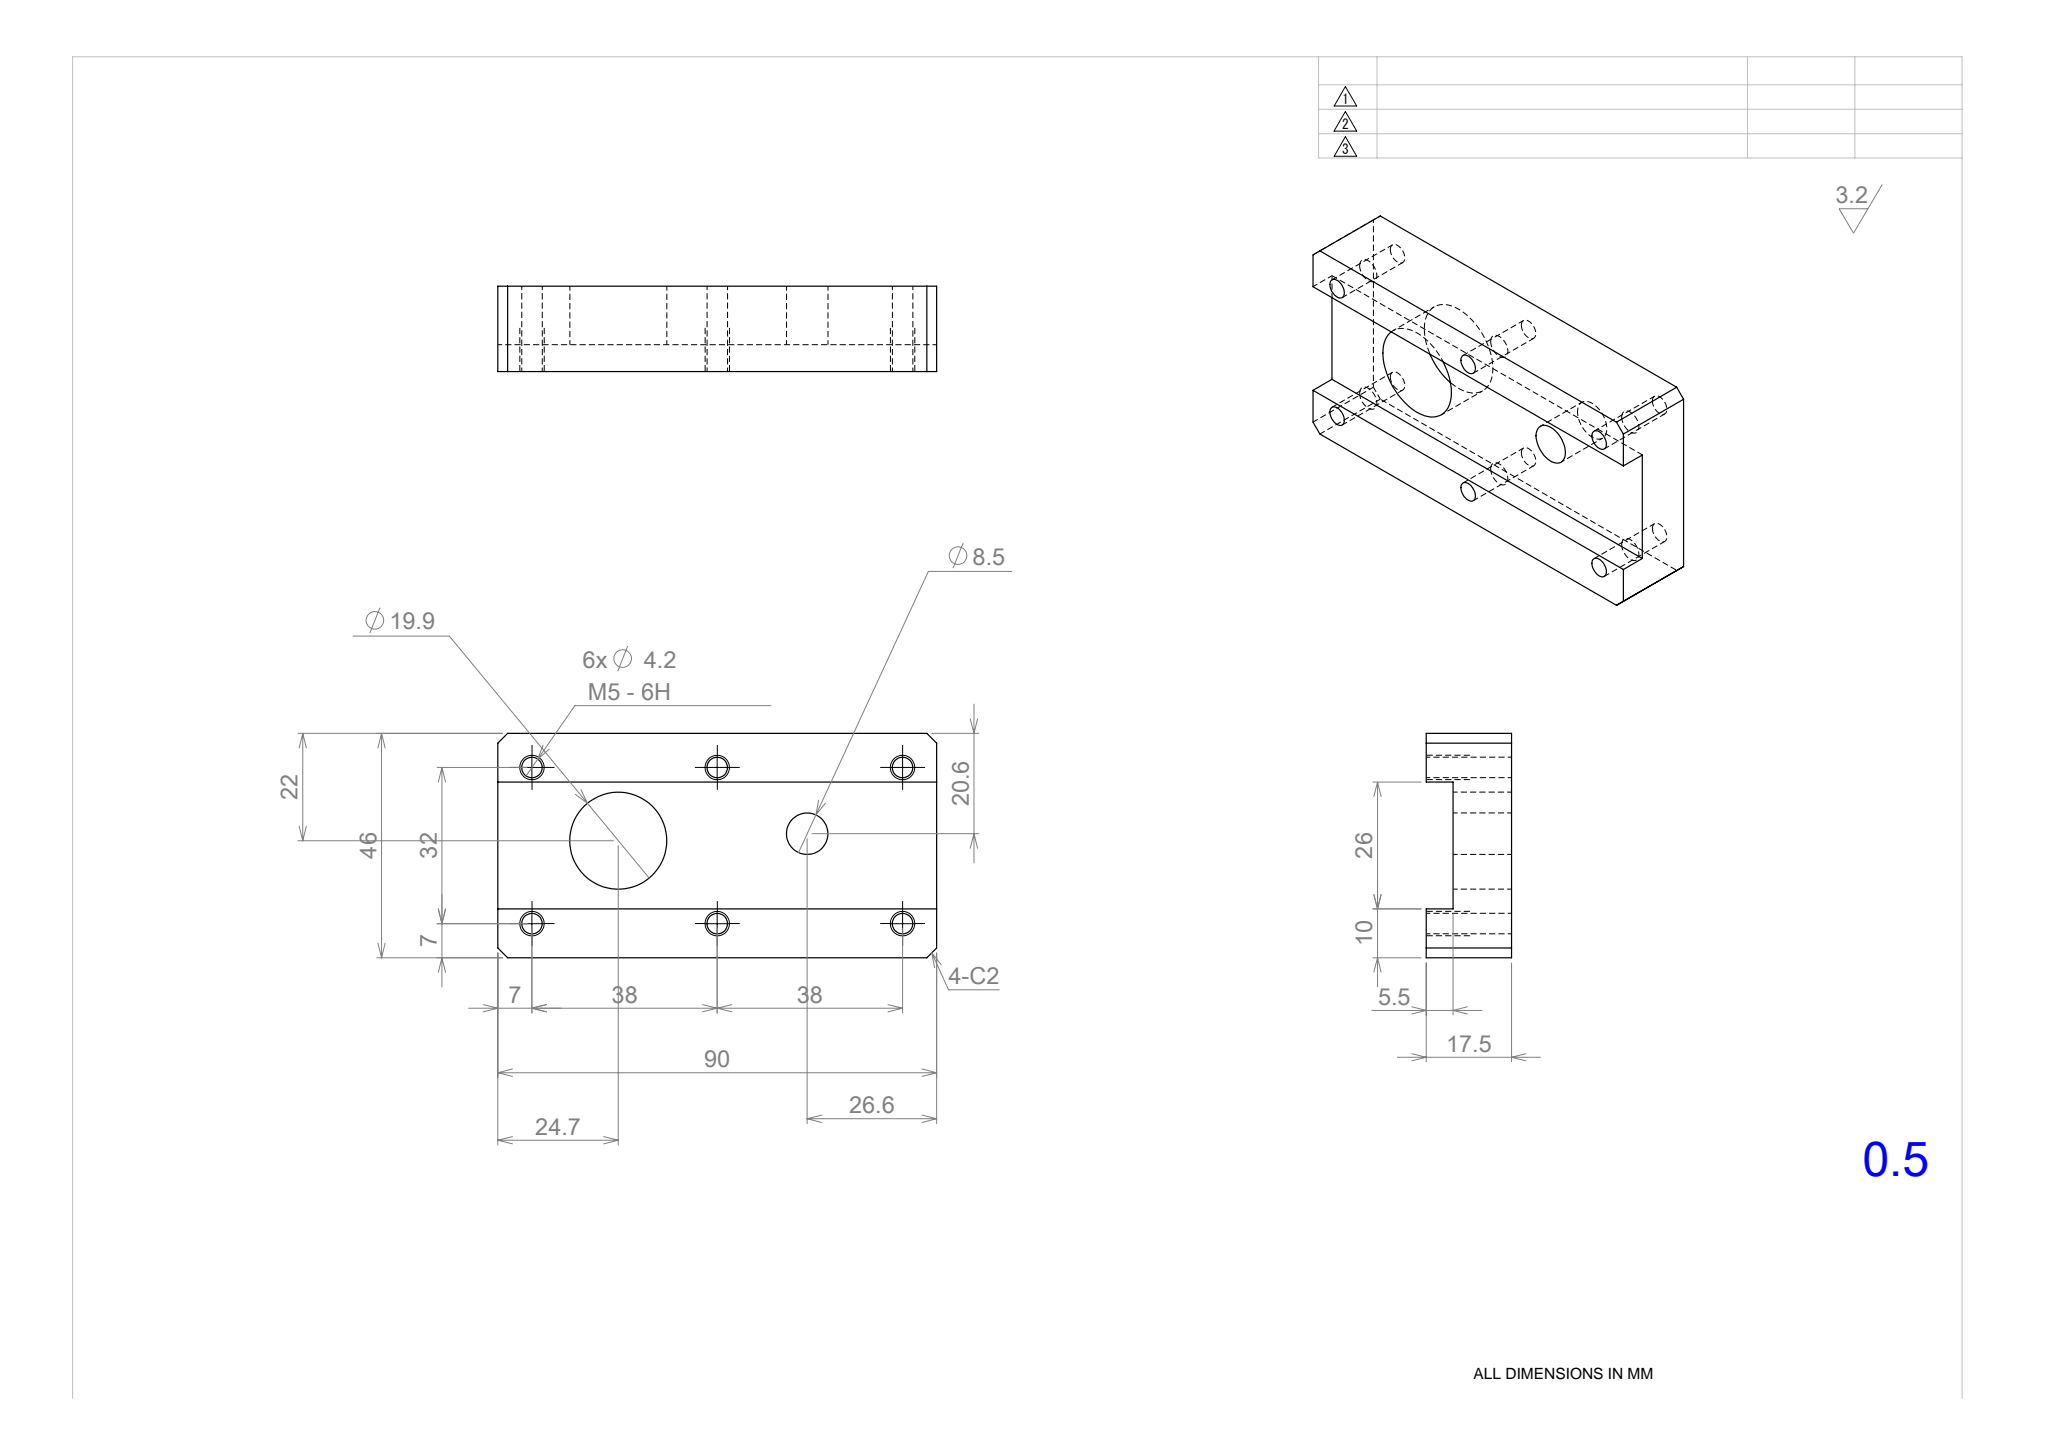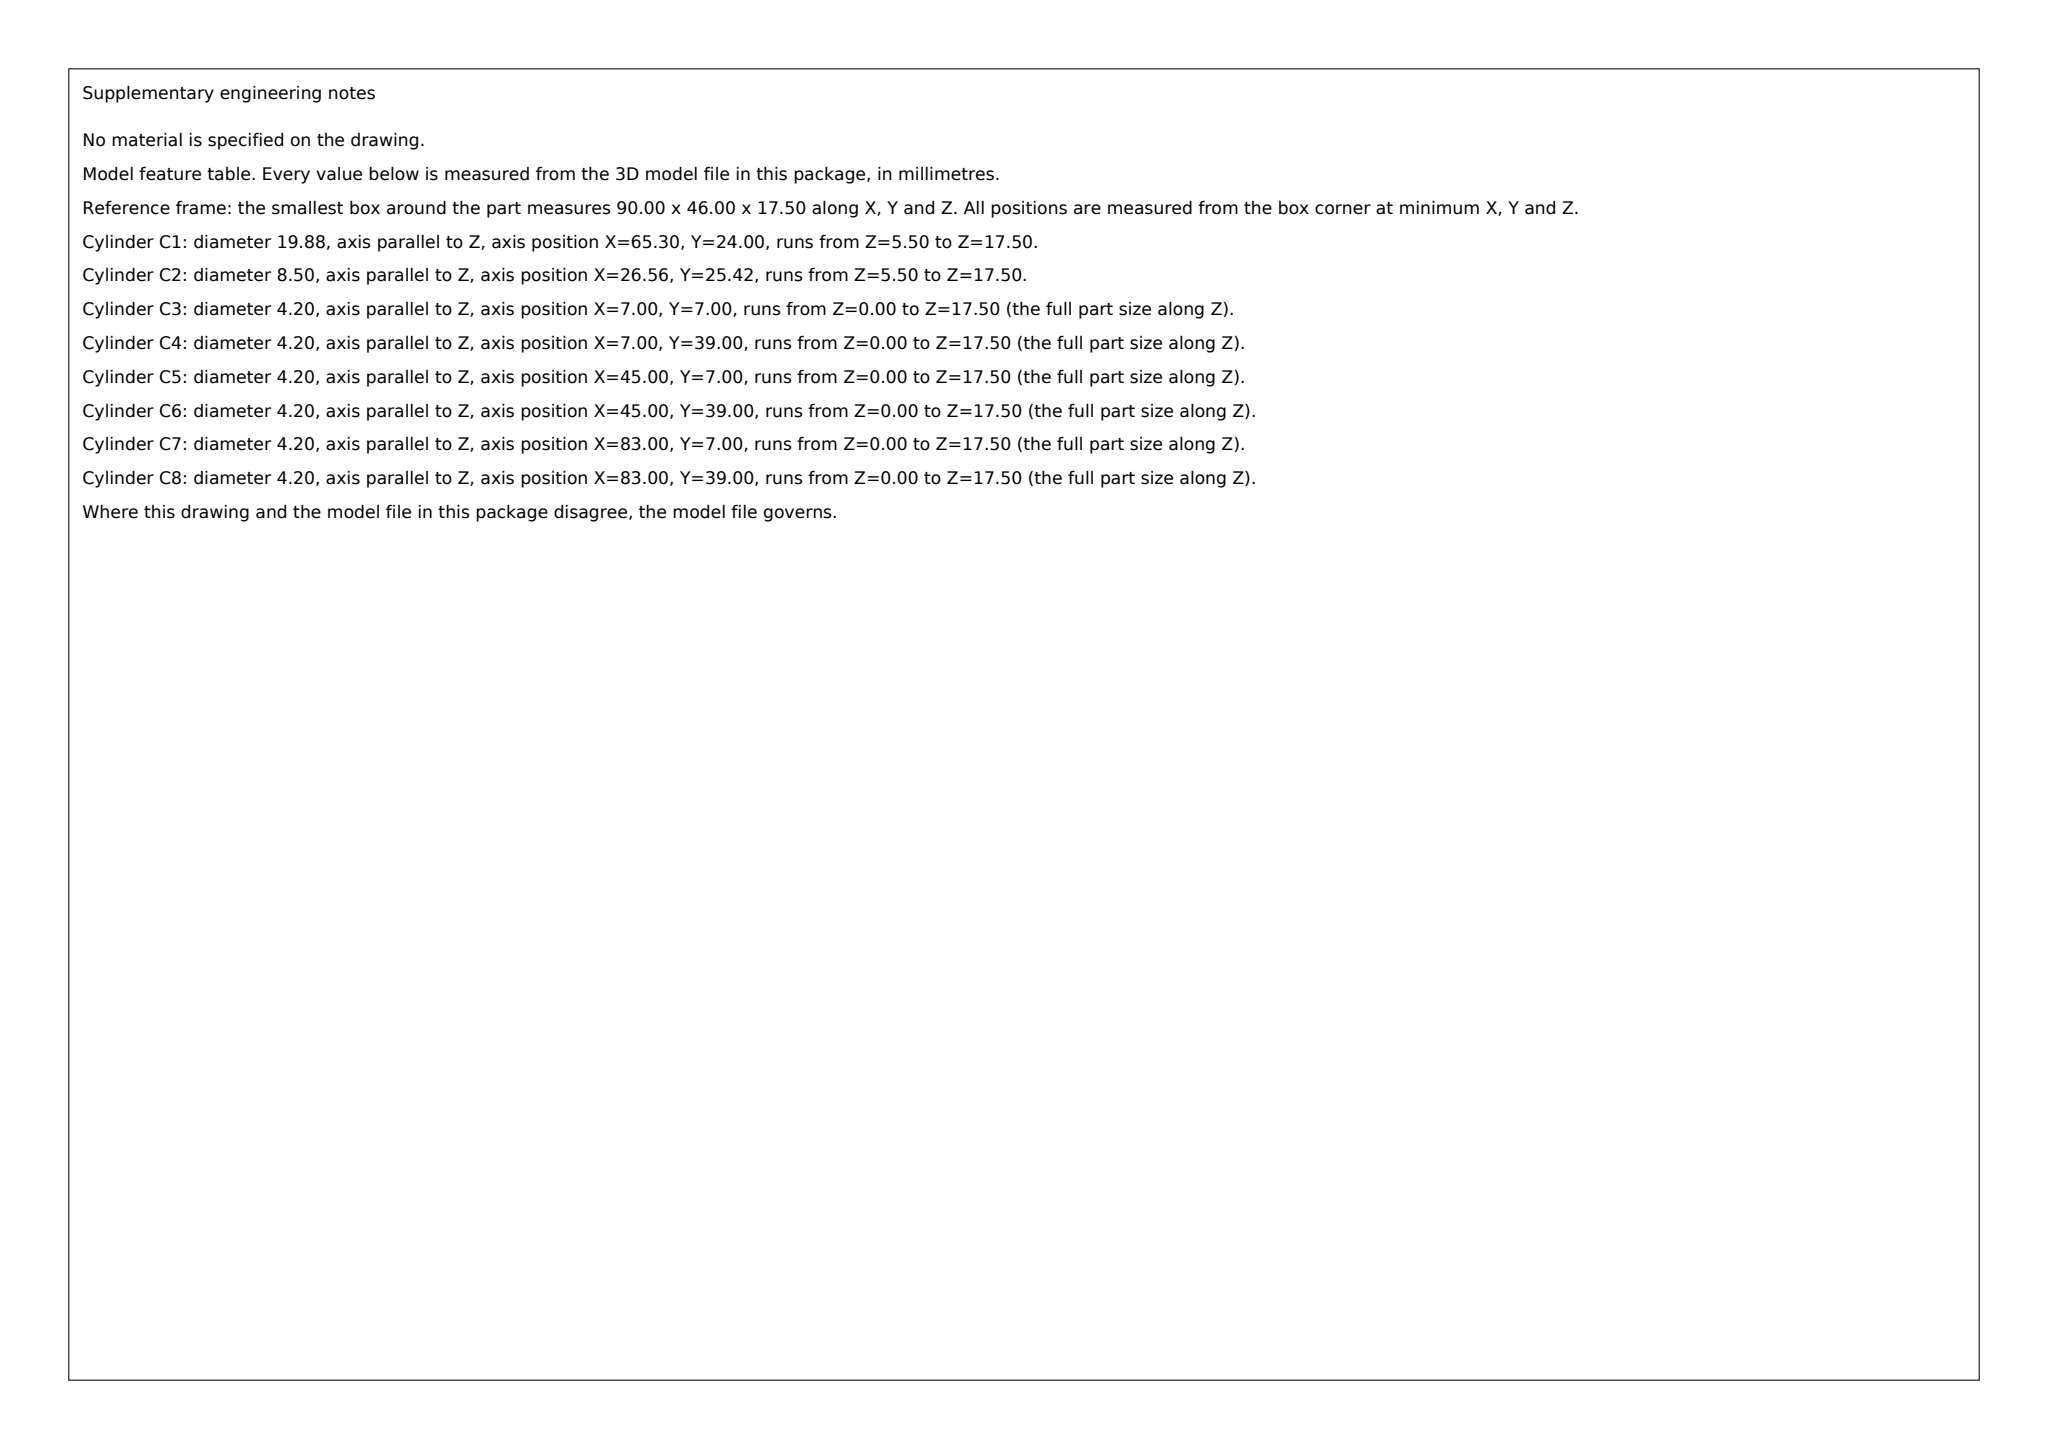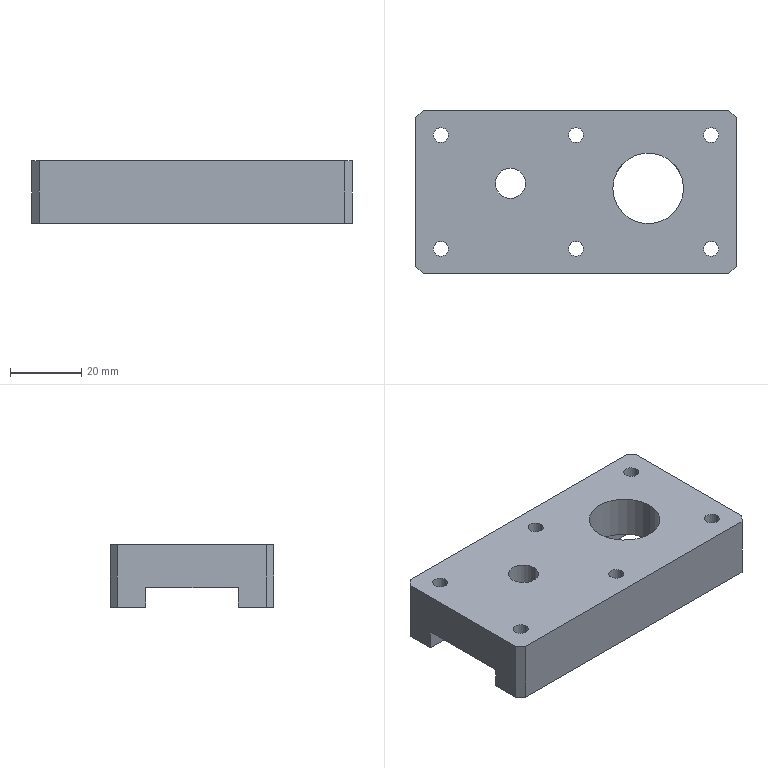Part | SolidWorks | mm | 1 solid | 30 faces | box 90 x 46 x 17.5 mm | volume 53578 mm3 | cylinder 16 | plane 14 | commonest cylinder face diameters 4.2 x12 8.498 x2 19.884 x2